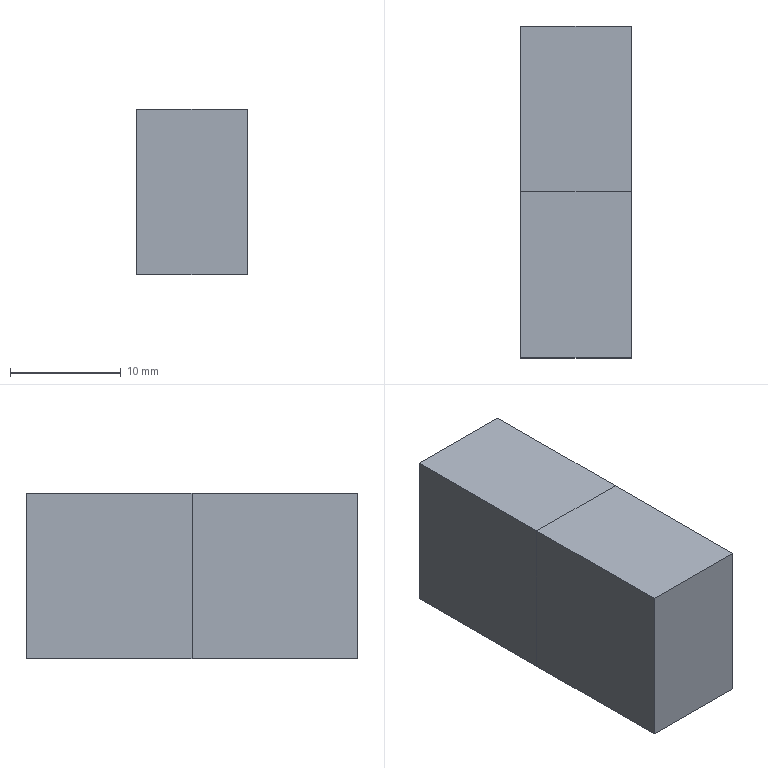Component | NX | 11_OBJECT | 2 solids | 12 faces | box 10 x 30 x 15 mm | volume 4500 mm3 | plane 12
STEP:
#1=CARTESIAN_POINT('',(0.,0.,0.));
#2=DIRECTION('',(0.,0.,1.));
#3=DIRECTION('',(1.,0.,0.));
#4=AXIS2_PLACEMENT_3D('',#1,#2,#3);
#5=CARTESIAN_POINT('',(2050.,126.,562.5));
#6=VERTEX_POINT('',#5);
#7=CARTESIAN_POINT('',(2050.,141.,562.5));
#8=VERTEX_POINT('',#7);
#9=CARTESIAN_POINT('',(2050.,126.,562.5));
#10=DIRECTION('',(0.,1.,0.));
#11=VECTOR('',#10,1.);
#12=LINE('',#9,#11);
#13=CARTESIAN_POINT('',(2060.,126.,562.5));
#14=DIRECTION('',(0.,0.,1.));
#15=DIRECTION('',(0.,1.,0.));
#16=AXIS2_PLACEMENT_3D('',#13,#14,#15);
#17=PLANE('',#16);
#18=CARTESIAN_POINT('',(0.,10.));
#19=DIRECTION('',(1.,0.));
#20=VECTOR('',#19,1.);
#21=LINE('',#18,#20);
#22=(GEOMETRIC_REPRESENTATION_CONTEXT(2)PARAMETRIC_REPRESENTATION_CONTEXT()REPRESENTATION_CONTEXT('',''));
#23=DEFINITIONAL_REPRESENTATION('',(#21),#22);
#24=PCURVE('',#17,#23);
#25=CARTESIAN_POINT('',(2050.,126.,562.5));
#26=DIRECTION('',(1.,0.,0.));
#27=DIRECTION('',(0.,1.,0.));
#28=AXIS2_PLACEMENT_3D('',#25,#26,#27);
#29=PLANE('',#28);
#30=CARTESIAN_POINT('',(0.,0.));
#31=DIRECTION('',(1.,0.));
#32=VECTOR('',#31,1.);
#33=LINE('',#30,#32);
#34=(GEOMETRIC_REPRESENTATION_CONTEXT(2)PARAMETRIC_REPRESENTATION_CONTEXT()REPRESENTATION_CONTEXT('',''));
#35=DEFINITIONAL_REPRESENTATION('',(#33),#34);
#36=PCURVE('',#29,#35);
#37=SURFACE_CURVE('',#12,(#24,#36),.PCURVE_S1.);
#38=EDGE_CURVE('',#6,#8,#37,.T.);
#39=ORIENTED_EDGE('',*,*,#38,.T.);
#40=CARTESIAN_POINT('',(2060.,141.,562.5));
#41=VERTEX_POINT('',#40);
#42=CARTESIAN_POINT('',(2060.,141.,562.5));
#43=DIRECTION('',(-1.,0.,0.));
#44=VECTOR('',#43,1.);
#45=LINE('',#42,#44);
#46=CARTESIAN_POINT('',(15.,0.));
#47=DIRECTION('',(0.,1.));
#48=VECTOR('',#47,1.);
#49=LINE('',#46,#48);
#50=(GEOMETRIC_REPRESENTATION_CONTEXT(2)PARAMETRIC_REPRESENTATION_CONTEXT()REPRESENTATION_CONTEXT('',''));
#51=DEFINITIONAL_REPRESENTATION('',(#49),#50);
#52=PCURVE('',#17,#51);
#53=CARTESIAN_POINT('',(2060.,141.,562.5));
#54=DIRECTION('',(0.,-1.,0.));
#55=DIRECTION('',(0.,0.,1.));
#56=AXIS2_PLACEMENT_3D('',#53,#54,#55);
#57=PLANE('',#56);
#58=CARTESIAN_POINT('',(0.,0.));
#59=DIRECTION('',(0.,1.));
#60=VECTOR('',#59,1.);
#61=LINE('',#58,#60);
#62=(GEOMETRIC_REPRESENTATION_CONTEXT(2)PARAMETRIC_REPRESENTATION_CONTEXT()REPRESENTATION_CONTEXT('',''));
#63=DEFINITIONAL_REPRESENTATION('',(#61),#62);
#64=PCURVE('',#57,#63);
#65=SURFACE_CURVE('',#45,(#52,#64),.PCURVE_S1.);
#66=EDGE_CURVE('',#41,#8,#65,.T.);
#67=ORIENTED_EDGE('',*,*,#66,.F.);
#68=CARTESIAN_POINT('',(2060.,126.,562.5));
#69=VERTEX_POINT('',#68);
#70=CARTESIAN_POINT('',(2060.,126.,562.5));
#71=DIRECTION('',(0.,1.,0.));
#72=VECTOR('',#71,1.);
#73=LINE('',#70,#72);
#74=CARTESIAN_POINT('',(0.,0.));
#75=DIRECTION('',(1.,0.));
#76=VECTOR('',#75,1.);
#77=LINE('',#74,#76);
#78=(GEOMETRIC_REPRESENTATION_CONTEXT(2)PARAMETRIC_REPRESENTATION_CONTEXT()REPRESENTATION_CONTEXT('',''));
#79=DEFINITIONAL_REPRESENTATION('',(#77),#78);
#80=PCURVE('',#17,#79);
#81=CARTESIAN_POINT('',(2060.,126.,562.5));
#82=DIRECTION('',(1.,0.,0.));
#83=DIRECTION('',(0.,1.,0.));
#84=AXIS2_PLACEMENT_3D('',#81,#82,#83);
#85=PLANE('',#84);
#86=CARTESIAN_POINT('',(0.,0.));
#87=DIRECTION('',(1.,0.));
#88=VECTOR('',#87,1.);
#89=LINE('',#86,#88);
#90=(GEOMETRIC_REPRESENTATION_CONTEXT(2)PARAMETRIC_REPRESENTATION_CONTEXT()REPRESENTATION_CONTEXT('',''));
#91=DEFINITIONAL_REPRESENTATION('',(#89),#90);
#92=PCURVE('',#85,#91);
#93=SURFACE_CURVE('',#73,(#80,#92),.PCURVE_S1.);
#94=EDGE_CURVE('',#69,#41,#93,.T.);
#95=ORIENTED_EDGE('',*,*,#94,.F.);
#96=CARTESIAN_POINT('',(2060.,126.,562.5));
#97=DIRECTION('',(-1.,0.,0.));
#98=VECTOR('',#97,1.);
#99=LINE('',#96,#98);
#100=CARTESIAN_POINT('',(0.,0.));
#101=DIRECTION('',(0.,1.));
#102=VECTOR('',#101,1.);
#103=LINE('',#100,#102);
#104=(GEOMETRIC_REPRESENTATION_CONTEXT(2)PARAMETRIC_REPRESENTATION_CONTEXT()REPRESENTATION_CONTEXT('',''));
#105=DEFINITIONAL_REPRESENTATION('',(#103),#104);
#106=PCURVE('',#17,#105);
#107=CARTESIAN_POINT('',(2060.,126.,577.5));
#108=DIRECTION('',(0.,1.,0.));
#109=DIRECTION('',(0.,0.,-1.));
#110=AXIS2_PLACEMENT_3D('',#107,#108,#109);
#111=PLANE('',#110);
#112=CARTESIAN_POINT('',(15.,0.));
#113=DIRECTION('',(0.,1.));
#114=VECTOR('',#113,1.);
#115=LINE('',#112,#114);
#116=(GEOMETRIC_REPRESENTATION_CONTEXT(2)PARAMETRIC_REPRESENTATION_CONTEXT()REPRESENTATION_CONTEXT('',''));
#117=DEFINITIONAL_REPRESENTATION('',(#115),#116);
#118=PCURVE('',#111,#117);
#119=SURFACE_CURVE('',#99,(#106,#118),.PCURVE_S1.);
#120=EDGE_CURVE('',#69,#6,#119,.T.);
#121=ORIENTED_EDGE('',*,*,#120,.T.);
#122=EDGE_LOOP('',(#39,#67,#95,#121));
#123=FACE_BOUND('',#122,.T.);
#124=ADVANCED_FACE('',(#123),#17,.F.);
#125=CARTESIAN_POINT('',(2050.,141.,577.5));
#126=VERTEX_POINT('',#125);
#127=CARTESIAN_POINT('',(2050.,141.,562.5));
#128=DIRECTION('',(0.,0.,1.));
#129=VECTOR('',#128,1.);
#130=LINE('',#127,#129);
#131=CARTESIAN_POINT('',(0.,10.));
#132=DIRECTION('',(1.,0.));
#133=VECTOR('',#132,1.);
#134=LINE('',#131,#133);
#135=(GEOMETRIC_REPRESENTATION_CONTEXT(2)PARAMETRIC_REPRESENTATION_CONTEXT()REPRESENTATION_CONTEXT('',''));
#136=DEFINITIONAL_REPRESENTATION('',(#134),#135);
#137=PCURVE('',#57,#136);
#138=CARTESIAN_POINT('',(15.,0.));
#139=DIRECTION('',(0.,1.));
#140=VECTOR('',#139,1.);
#141=LINE('',#138,#140);
#142=(GEOMETRIC_REPRESENTATION_CONTEXT(2)PARAMETRIC_REPRESENTATION_CONTEXT()REPRESENTATION_CONTEXT('',''));
#143=DEFINITIONAL_REPRESENTATION('',(#141),#142);
#144=PCURVE('',#29,#143);
#145=SURFACE_CURVE('',#130,(#137,#144),.PCURVE_S1.);
#146=EDGE_CURVE('',#8,#126,#145,.T.);
#147=ORIENTED_EDGE('',*,*,#146,.T.);
#148=CARTESIAN_POINT('',(2060.,141.,577.5));
#149=VERTEX_POINT('',#148);
#150=CARTESIAN_POINT('',(2060.,141.,577.5));
#151=DIRECTION('',(-1.,0.,0.));
#152=VECTOR('',#151,1.);
#153=LINE('',#150,#152);
#154=CARTESIAN_POINT('',(15.,0.));
#155=DIRECTION('',(0.,1.));
#156=VECTOR('',#155,1.);
#157=LINE('',#154,#156);
#158=(GEOMETRIC_REPRESENTATION_CONTEXT(2)PARAMETRIC_REPRESENTATION_CONTEXT()REPRESENTATION_CONTEXT('',''));
#159=DEFINITIONAL_REPRESENTATION('',(#157),#158);
#160=PCURVE('',#57,#159);
#161=CARTESIAN_POINT('',(2060.,141.,577.5));
#162=DIRECTION('',(0.,0.,-1.));
#163=DIRECTION('',(0.,-1.,0.));
#164=AXIS2_PLACEMENT_3D('',#161,#162,#163);
#165=PLANE('',#164);
#166=CARTESIAN_POINT('',(0.,0.));
#167=DIRECTION('',(0.,1.));
#168=VECTOR('',#167,1.);
#169=LINE('',#166,#168);
#170=(GEOMETRIC_REPRESENTATION_CONTEXT(2)PARAMETRIC_REPRESENTATION_CONTEXT()REPRESENTATION_CONTEXT('',''));
#171=DEFINITIONAL_REPRESENTATION('',(#169),#170);
#172=PCURVE('',#165,#171);
#173=SURFACE_CURVE('',#153,(#160,#172),.PCURVE_S1.);
#174=EDGE_CURVE('',#149,#126,#173,.T.);
#175=ORIENTED_EDGE('',*,*,#174,.F.);
#176=CARTESIAN_POINT('',(2060.,141.,562.5));
#177=DIRECTION('',(0.,0.,1.));
#178=VECTOR('',#177,1.);
#179=LINE('',#176,#178);
#180=CARTESIAN_POINT('',(0.,0.));
#181=DIRECTION('',(1.,0.));
#182=VECTOR('',#181,1.);
#183=LINE('',#180,#182);
#184=(GEOMETRIC_REPRESENTATION_CONTEXT(2)PARAMETRIC_REPRESENTATION_CONTEXT()REPRESENTATION_CONTEXT('',''));
#185=DEFINITIONAL_REPRESENTATION('',(#183),#184);
#186=PCURVE('',#57,#185);
#187=CARTESIAN_POINT('',(15.,0.));
#188=DIRECTION('',(0.,1.));
#189=VECTOR('',#188,1.);
#190=LINE('',#187,#189);
#191=(GEOMETRIC_REPRESENTATION_CONTEXT(2)PARAMETRIC_REPRESENTATION_CONTEXT()REPRESENTATION_CONTEXT('',''));
#192=DEFINITIONAL_REPRESENTATION('',(#190),#191);
#193=PCURVE('',#85,#192);
#194=SURFACE_CURVE('',#179,(#186,#193),.PCURVE_S1.);
#195=EDGE_CURVE('',#41,#149,#194,.T.);
#196=ORIENTED_EDGE('',*,*,#195,.F.);
#197=ORIENTED_EDGE('',*,*,#66,.T.);
#198=EDGE_LOOP('',(#147,#175,#196,#197));
#199=FACE_BOUND('',#198,.T.);
#200=ADVANCED_FACE('',(#199),#57,.F.);
#201=CARTESIAN_POINT('',(2050.,126.,577.5));
#202=VERTEX_POINT('',#201);
#203=CARTESIAN_POINT('',(2050.,141.,577.5));
#204=DIRECTION('',(0.,-1.,0.));
#205=VECTOR('',#204,1.);
#206=LINE('',#203,#205);
#207=CARTESIAN_POINT('',(0.,10.));
#208=DIRECTION('',(1.,0.));
#209=VECTOR('',#208,1.);
#210=LINE('',#207,#209);
#211=(GEOMETRIC_REPRESENTATION_CONTEXT(2)PARAMETRIC_REPRESENTATION_CONTEXT()REPRESENTATION_CONTEXT('',''));
#212=DEFINITIONAL_REPRESENTATION('',(#210),#211);
#213=PCURVE('',#165,#212);
#214=CARTESIAN_POINT('',(15.,15.));
#215=DIRECTION('',(-1.,0.));
#216=VECTOR('',#215,1.);
#217=LINE('',#214,#216);
#218=(GEOMETRIC_REPRESENTATION_CONTEXT(2)PARAMETRIC_REPRESENTATION_CONTEXT()REPRESENTATION_CONTEXT('',''));
#219=DEFINITIONAL_REPRESENTATION('',(#217),#218);
#220=PCURVE('',#29,#219);
#221=SURFACE_CURVE('',#206,(#213,#220),.PCURVE_S1.);
#222=EDGE_CURVE('',#126,#202,#221,.T.);
#223=ORIENTED_EDGE('',*,*,#222,.T.);
#224=CARTESIAN_POINT('',(2060.,126.,577.5));
#225=VERTEX_POINT('',#224);
#226=CARTESIAN_POINT('',(2060.,126.,577.5));
#227=DIRECTION('',(-1.,0.,0.));
#228=VECTOR('',#227,1.);
#229=LINE('',#226,#228);
#230=CARTESIAN_POINT('',(15.,0.));
#231=DIRECTION('',(0.,1.));
#232=VECTOR('',#231,1.);
#233=LINE('',#230,#232);
#234=(GEOMETRIC_REPRESENTATION_CONTEXT(2)PARAMETRIC_REPRESENTATION_CONTEXT()REPRESENTATION_CONTEXT('',''));
#235=DEFINITIONAL_REPRESENTATION('',(#233),#234);
#236=PCURVE('',#165,#235);
#237=CARTESIAN_POINT('',(0.,0.));
#238=DIRECTION('',(0.,1.));
#239=VECTOR('',#238,1.);
#240=LINE('',#237,#239);
#241=(GEOMETRIC_REPRESENTATION_CONTEXT(2)PARAMETRIC_REPRESENTATION_CONTEXT()REPRESENTATION_CONTEXT('',''));
#242=DEFINITIONAL_REPRESENTATION('',(#240),#241);
#243=PCURVE('',#111,#242);
#244=SURFACE_CURVE('',#229,(#236,#243),.PCURVE_S1.);
#245=EDGE_CURVE('',#225,#202,#244,.T.);
#246=ORIENTED_EDGE('',*,*,#245,.F.);
#247=CARTESIAN_POINT('',(2060.,141.,577.5));
#248=DIRECTION('',(0.,-1.,0.));
#249=VECTOR('',#248,1.);
#250=LINE('',#247,#249);
#251=CARTESIAN_POINT('',(0.,0.));
#252=DIRECTION('',(1.,0.));
#253=VECTOR('',#252,1.);
#254=LINE('',#251,#253);
#255=(GEOMETRIC_REPRESENTATION_CONTEXT(2)PARAMETRIC_REPRESENTATION_CONTEXT()REPRESENTATION_CONTEXT('',''));
#256=DEFINITIONAL_REPRESENTATION('',(#254),#255);
#257=PCURVE('',#165,#256);
#258=CARTESIAN_POINT('',(15.,15.));
#259=DIRECTION('',(-1.,0.));
#260=VECTOR('',#259,1.);
#261=LINE('',#258,#260);
#262=(GEOMETRIC_REPRESENTATION_CONTEXT(2)PARAMETRIC_REPRESENTATION_CONTEXT()REPRESENTATION_CONTEXT('',''));
#263=DEFINITIONAL_REPRESENTATION('',(#261),#262);
#264=PCURVE('',#85,#263);
#265=SURFACE_CURVE('',#250,(#257,#264),.PCURVE_S1.);
#266=EDGE_CURVE('',#149,#225,#265,.T.);
#267=ORIENTED_EDGE('',*,*,#266,.F.);
#268=ORIENTED_EDGE('',*,*,#174,.T.);
#269=EDGE_LOOP('',(#223,#246,#267,#268));
#270=FACE_BOUND('',#269,.T.);
#271=ADVANCED_FACE('',(#270),#165,.F.);
#272=CARTESIAN_POINT('',(2050.,126.,577.5));
#273=DIRECTION('',(0.,0.,-1.));
#274=VECTOR('',#273,1.);
#275=LINE('',#272,#274);
#276=CARTESIAN_POINT('',(0.,10.));
#277=DIRECTION('',(1.,0.));
#278=VECTOR('',#277,1.);
#279=LINE('',#276,#278);
#280=(GEOMETRIC_REPRESENTATION_CONTEXT(2)PARAMETRIC_REPRESENTATION_CONTEXT()REPRESENTATION_CONTEXT('',''));
#281=DEFINITIONAL_REPRESENTATION('',(#279),#280);
#282=PCURVE('',#111,#281);
#283=CARTESIAN_POINT('',(0.,15.));
#284=DIRECTION('',(0.,-1.));
#285=VECTOR('',#284,1.);
#286=LINE('',#283,#285);
#287=(GEOMETRIC_REPRESENTATION_CONTEXT(2)PARAMETRIC_REPRESENTATION_CONTEXT()REPRESENTATION_CONTEXT('',''));
#288=DEFINITIONAL_REPRESENTATION('',(#286),#287);
#289=PCURVE('',#29,#288);
#290=SURFACE_CURVE('',#275,(#282,#289),.PCURVE_S1.);
#291=EDGE_CURVE('',#202,#6,#290,.T.);
#292=ORIENTED_EDGE('',*,*,#291,.T.);
#293=ORIENTED_EDGE('',*,*,#120,.F.);
#294=CARTESIAN_POINT('',(2060.,126.,577.5));
#295=DIRECTION('',(0.,0.,-1.));
#296=VECTOR('',#295,1.);
#297=LINE('',#294,#296);
#298=CARTESIAN_POINT('',(0.,0.));
#299=DIRECTION('',(1.,0.));
#300=VECTOR('',#299,1.);
#301=LINE('',#298,#300);
#302=(GEOMETRIC_REPRESENTATION_CONTEXT(2)PARAMETRIC_REPRESENTATION_CONTEXT()REPRESENTATION_CONTEXT('',''));
#303=DEFINITIONAL_REPRESENTATION('',(#301),#302);
#304=PCURVE('',#111,#303);
#305=CARTESIAN_POINT('',(0.,15.));
#306=DIRECTION('',(0.,-1.));
#307=VECTOR('',#306,1.);
#308=LINE('',#305,#307);
#309=(GEOMETRIC_REPRESENTATION_CONTEXT(2)PARAMETRIC_REPRESENTATION_CONTEXT()REPRESENTATION_CONTEXT('',''));
#310=DEFINITIONAL_REPRESENTATION('',(#308),#309);
#311=PCURVE('',#85,#310);
#312=SURFACE_CURVE('',#297,(#304,#311),.PCURVE_S1.);
#313=EDGE_CURVE('',#225,#69,#312,.T.);
#314=ORIENTED_EDGE('',*,*,#313,.F.);
#315=ORIENTED_EDGE('',*,*,#245,.T.);
#316=EDGE_LOOP('',(#292,#293,#314,#315));
#317=FACE_BOUND('',#316,.T.);
#318=ADVANCED_FACE('',(#317),#111,.F.);
#319=ORIENTED_EDGE('',*,*,#94,.T.);
#320=ORIENTED_EDGE('',*,*,#195,.T.);
#321=ORIENTED_EDGE('',*,*,#266,.T.);
#322=ORIENTED_EDGE('',*,*,#313,.T.);
#323=EDGE_LOOP('',(#319,#320,#321,#322));
#324=FACE_BOUND('',#323,.T.);
#325=ADVANCED_FACE('',(#324),#85,.T.);
#326=ORIENTED_EDGE('',*,*,#38,.F.);
#327=ORIENTED_EDGE('',*,*,#291,.F.);
#328=ORIENTED_EDGE('',*,*,#222,.F.);
#329=ORIENTED_EDGE('',*,*,#146,.F.);
#330=EDGE_LOOP('',(#326,#327,#328,#329));
#331=FACE_BOUND('',#330,.T.);
#332=ADVANCED_FACE('',(#331),#29,.F.);
#333=CLOSED_SHELL('',(#124,#200,#271,#318,#325,#332));
#334=MANIFOLD_SOLID_BREP('',#333);
#335=(LENGTH_UNIT()NAMED_UNIT(*)SI_UNIT(.MILLI.,.METRE.));
#336=UNCERTAINTY_MEASURE_WITH_UNIT(LENGTH_MEASURE(0.0000001),#335,'','');
#337=(NAMED_UNIT(*)PLANE_ANGLE_UNIT()SI_UNIT($,.RADIAN.));
#338=(NAMED_UNIT(*)SI_UNIT($,.STERADIAN.)SOLID_ANGLE_UNIT());
#339=(GEOMETRIC_REPRESENTATION_CONTEXT(3)GLOBAL_UNCERTAINTY_ASSIGNED_CONTEXT((#336))GLOBAL_UNIT_ASSIGNED_CONTEXT((#335,#337,#338))REPRESENTATION_CONTEXT('',''));
#340=ADVANCED_BREP_SHAPE_REPRESENTATION('',(#4,#334),#339);
#341=CARTESIAN_POINT('',(0.,0.,0.));
#342=DIRECTION('',(0.,0.,1.));
#343=DIRECTION('',(1.,0.,0.));
#344=AXIS2_PLACEMENT_3D('',#341,#342,#343);
#345=CARTESIAN_POINT('',(0.,0.,0.));
#346=DIRECTION('',(0.,0.,1.));
#347=DIRECTION('',(1.,0.,0.));
#348=AXIS2_PLACEMENT_3D('',#345,#346,#347);
#349=(LENGTH_UNIT()NAMED_UNIT(*)SI_UNIT(.MILLI.,.METRE.));
#350=UNCERTAINTY_MEASURE_WITH_UNIT(LENGTH_MEASURE(0.0000001),#349,'','');
#351=(NAMED_UNIT(*)PLANE_ANGLE_UNIT()SI_UNIT($,.RADIAN.));
#352=(NAMED_UNIT(*)SI_UNIT($,.STERADIAN.)SOLID_ANGLE_UNIT());
#353=(GEOMETRIC_REPRESENTATION_CONTEXT(3)GLOBAL_UNCERTAINTY_ASSIGNED_CONTEXT((#350))GLOBAL_UNIT_ASSIGNED_CONTEXT((#349,#351,#352))REPRESENTATION_CONTEXT('',''));
#354=SHAPE_REPRESENTATION('',(#4,#344,#348),#353);
#355=ITEM_DEFINED_TRANSFORMATION('','',#4,#344);
#356=(REPRESENTATION_RELATIONSHIP('','',#340,#354)REPRESENTATION_RELATIONSHIP_WITH_TRANSFORMATION(#355)SHAPE_REPRESENTATION_RELATIONSHIP());
#357=CARTESIAN_POINT('',(2050.,111.,562.5));
#358=VERTEX_POINT('',#357);
#359=CARTESIAN_POINT('',(2050.,126.,562.5));
#360=VERTEX_POINT('',#359);
#361=CARTESIAN_POINT('',(2050.,111.,562.5));
#362=DIRECTION('',(0.,1.,0.));
#363=VECTOR('',#362,1.);
#364=LINE('',#361,#363);
#365=CARTESIAN_POINT('',(2060.,111.,562.5));
#366=DIRECTION('',(0.,0.,1.));
#367=DIRECTION('',(0.,1.,0.));
#368=AXIS2_PLACEMENT_3D('',#365,#366,#367);
#369=PLANE('',#368);
#370=CARTESIAN_POINT('',(0.,10.));
#371=DIRECTION('',(1.,0.));
#372=VECTOR('',#371,1.);
#373=LINE('',#370,#372);
#374=(GEOMETRIC_REPRESENTATION_CONTEXT(2)PARAMETRIC_REPRESENTATION_CONTEXT()REPRESENTATION_CONTEXT('',''));
#375=DEFINITIONAL_REPRESENTATION('',(#373),#374);
#376=PCURVE('',#369,#375);
#377=CARTESIAN_POINT('',(2050.,111.,562.5));
#378=DIRECTION('',(1.,0.,0.));
#379=DIRECTION('',(0.,1.,0.));
#380=AXIS2_PLACEMENT_3D('',#377,#378,#379);
#381=PLANE('',#380);
#382=CARTESIAN_POINT('',(0.,0.));
#383=DIRECTION('',(1.,0.));
#384=VECTOR('',#383,1.);
#385=LINE('',#382,#384);
#386=(GEOMETRIC_REPRESENTATION_CONTEXT(2)PARAMETRIC_REPRESENTATION_CONTEXT()REPRESENTATION_CONTEXT('',''));
#387=DEFINITIONAL_REPRESENTATION('',(#385),#386);
#388=PCURVE('',#381,#387);
#389=SURFACE_CURVE('',#364,(#376,#388),.PCURVE_S1.);
#390=EDGE_CURVE('',#358,#360,#389,.T.);
#391=ORIENTED_EDGE('',*,*,#390,.T.);
#392=CARTESIAN_POINT('',(2060.,126.,562.5));
#393=VERTEX_POINT('',#392);
#394=CARTESIAN_POINT('',(2060.,126.,562.5));
#395=DIRECTION('',(-1.,0.,0.));
#396=VECTOR('',#395,1.);
#397=LINE('',#394,#396);
#398=CARTESIAN_POINT('',(15.,0.));
#399=DIRECTION('',(0.,1.));
#400=VECTOR('',#399,1.);
#401=LINE('',#398,#400);
#402=(GEOMETRIC_REPRESENTATION_CONTEXT(2)PARAMETRIC_REPRESENTATION_CONTEXT()REPRESENTATION_CONTEXT('',''));
#403=DEFINITIONAL_REPRESENTATION('',(#401),#402);
#404=PCURVE('',#369,#403);
#405=CARTESIAN_POINT('',(2060.,126.,562.5));
#406=DIRECTION('',(0.,-1.,0.));
#407=DIRECTION('',(0.,0.,1.));
#408=AXIS2_PLACEMENT_3D('',#405,#406,#407);
#409=PLANE('',#408);
#410=CARTESIAN_POINT('',(0.,0.));
#411=DIRECTION('',(0.,1.));
#412=VECTOR('',#411,1.);
#413=LINE('',#410,#412);
#414=(GEOMETRIC_REPRESENTATION_CONTEXT(2)PARAMETRIC_REPRESENTATION_CONTEXT()REPRESENTATION_CONTEXT('',''));
#415=DEFINITIONAL_REPRESENTATION('',(#413),#414);
#416=PCURVE('',#409,#415);
#417=SURFACE_CURVE('',#397,(#404,#416),.PCURVE_S1.);
#418=EDGE_CURVE('',#393,#360,#417,.T.);
#419=ORIENTED_EDGE('',*,*,#418,.F.);
#420=CARTESIAN_POINT('',(2060.,111.,562.5));
#421=VERTEX_POINT('',#420);
#422=CARTESIAN_POINT('',(2060.,111.,562.5));
#423=DIRECTION('',(0.,1.,0.));
#424=VECTOR('',#423,1.);
#425=LINE('',#422,#424);
#426=CARTESIAN_POINT('',(0.,0.));
#427=DIRECTION('',(1.,0.));
#428=VECTOR('',#427,1.);
#429=LINE('',#426,#428);
#430=(GEOMETRIC_REPRESENTATION_CONTEXT(2)PARAMETRIC_REPRESENTATION_CONTEXT()REPRESENTATION_CONTEXT('',''));
#431=DEFINITIONAL_REPRESENTATION('',(#429),#430);
#432=PCURVE('',#369,#431);
#433=CARTESIAN_POINT('',(2060.,111.,562.5));
#434=DIRECTION('',(1.,0.,0.));
#435=DIRECTION('',(0.,1.,0.));
#436=AXIS2_PLACEMENT_3D('',#433,#434,#435);
#437=PLANE('',#436);
#438=CARTESIAN_POINT('',(0.,0.));
#439=DIRECTION('',(1.,0.));
#440=VECTOR('',#439,1.);
#441=LINE('',#438,#440);
#442=(GEOMETRIC_REPRESENTATION_CONTEXT(2)PARAMETRIC_REPRESENTATION_CONTEXT()REPRESENTATION_CONTEXT('',''));
#443=DEFINITIONAL_REPRESENTATION('',(#441),#442);
#444=PCURVE('',#437,#443);
#445=SURFACE_CURVE('',#425,(#432,#444),.PCURVE_S1.);
#446=EDGE_CURVE('',#421,#393,#445,.T.);
#447=ORIENTED_EDGE('',*,*,#446,.F.);
#448=CARTESIAN_POINT('',(2060.,111.,562.5));
#449=DIRECTION('',(-1.,0.,0.));
#450=VECTOR('',#449,1.);
#451=LINE('',#448,#450);
#452=CARTESIAN_POINT('',(0.,0.));
#453=DIRECTION('',(0.,1.));
#454=VECTOR('',#453,1.);
#455=LINE('',#452,#454);
#456=(GEOMETRIC_REPRESENTATION_CONTEXT(2)PARAMETRIC_REPRESENTATION_CONTEXT()REPRESENTATION_CONTEXT('',''));
#457=DEFINITIONAL_REPRESENTATION('',(#455),#456);
#458=PCURVE('',#369,#457);
#459=CARTESIAN_POINT('',(2060.,111.,577.5));
#460=DIRECTION('',(0.,1.,0.));
#461=DIRECTION('',(0.,0.,-1.));
#462=AXIS2_PLACEMENT_3D('',#459,#460,#461);
#463=PLANE('',#462);
#464=CARTESIAN_POINT('',(15.,0.));
#465=DIRECTION('',(0.,1.));
#466=VECTOR('',#465,1.);
#467=LINE('',#464,#466);
#468=(GEOMETRIC_REPRESENTATION_CONTEXT(2)PARAMETRIC_REPRESENTATION_CONTEXT()REPRESENTATION_CONTEXT('',''));
#469=DEFINITIONAL_REPRESENTATION('',(#467),#468);
#470=PCURVE('',#463,#469);
#471=SURFACE_CURVE('',#451,(#458,#470),.PCURVE_S1.);
#472=EDGE_CURVE('',#421,#358,#471,.T.);
#473=ORIENTED_EDGE('',*,*,#472,.T.);
#474=EDGE_LOOP('',(#391,#419,#447,#473));
#475=FACE_BOUND('',#474,.T.);
#476=ADVANCED_FACE('',(#475),#369,.F.);
#477=CARTESIAN_POINT('',(2050.,126.,577.5));
#478=VERTEX_POINT('',#477);
#479=CARTESIAN_POINT('',(2050.,126.,562.5));
#480=DIRECTION('',(0.,0.,1.));
#481=VECTOR('',#480,1.);
#482=LINE('',#479,#481);
#483=CARTESIAN_POINT('',(0.,10.));
#484=DIRECTION('',(1.,0.));
#485=VECTOR('',#484,1.);
#486=LINE('',#483,#485);
#487=(GEOMETRIC_REPRESENTATION_CONTEXT(2)PARAMETRIC_REPRESENTATION_CONTEXT()REPRESENTATION_CONTEXT('',''));
#488=DEFINITIONAL_REPRESENTATION('',(#486),#487);
#489=PCURVE('',#409,#488);
#490=CARTESIAN_POINT('',(15.,0.));
#491=DIRECTION('',(0.,1.));
#492=VECTOR('',#491,1.);
#493=LINE('',#490,#492);
#494=(GEOMETRIC_REPRESENTATION_CONTEXT(2)PARAMETRIC_REPRESENTATION_CONTEXT()REPRESENTATION_CONTEXT('',''));
#495=DEFINITIONAL_REPRESENTATION('',(#493),#494);
#496=PCURVE('',#381,#495);
#497=SURFACE_CURVE('',#482,(#489,#496),.PCURVE_S1.);
#498=EDGE_CURVE('',#360,#478,#497,.T.);
#499=ORIENTED_EDGE('',*,*,#498,.T.);
#500=CARTESIAN_POINT('',(2060.,126.,577.5));
#501=VERTEX_POINT('',#500);
#502=CARTESIAN_POINT('',(2060.,126.,577.5));
#503=DIRECTION('',(-1.,0.,0.));
#504=VECTOR('',#503,1.);
#505=LINE('',#502,#504);
#506=CARTESIAN_POINT('',(15.,0.));
#507=DIRECTION('',(0.,1.));
#508=VECTOR('',#507,1.);
#509=LINE('',#506,#508);
#510=(GEOMETRIC_REPRESENTATION_CONTEXT(2)PARAMETRIC_REPRESENTATION_CONTEXT()REPRESENTATION_CONTEXT('',''));
#511=DEFINITIONAL_REPRESENTATION('',(#509),#510);
#512=PCURVE('',#409,#511);
#513=CARTESIAN_POINT('',(2060.,126.,577.5));
#514=DIRECTION('',(0.,0.,-1.));
#515=DIRECTION('',(0.,-1.,0.));
#516=AXIS2_PLACEMENT_3D('',#513,#514,#515);
#517=PLANE('',#516);
#518=CARTESIAN_POINT('',(0.,0.));
#519=DIRECTION('',(0.,1.));
#520=VECTOR('',#519,1.);
#521=LINE('',#518,#520);
#522=(GEOMETRIC_REPRESENTATION_CONTEXT(2)PARAMETRIC_REPRESENTATION_CONTEXT()REPRESENTATION_CONTEXT('',''));
#523=DEFINITIONAL_REPRESENTATION('',(#521),#522);
#524=PCURVE('',#517,#523);
#525=SURFACE_CURVE('',#505,(#512,#524),.PCURVE_S1.);
#526=EDGE_CURVE('',#501,#478,#525,.T.);
#527=ORIENTED_EDGE('',*,*,#526,.F.);
#528=CARTESIAN_POINT('',(2060.,126.,562.5));
#529=DIRECTION('',(0.,0.,1.));
#530=VECTOR('',#529,1.);
#531=LINE('',#528,#530);
#532=CARTESIAN_POINT('',(0.,0.));
#533=DIRECTION('',(1.,0.));
#534=VECTOR('',#533,1.);
#535=LINE('',#532,#534);
#536=(GEOMETRIC_REPRESENTATION_CONTEXT(2)PARAMETRIC_REPRESENTATION_CONTEXT()REPRESENTATION_CONTEXT('',''));
#537=DEFINITIONAL_REPRESENTATION('',(#535),#536);
#538=PCURVE('',#409,#537);
#539=CARTESIAN_POINT('',(15.,0.));
#540=DIRECTION('',(0.,1.));
#541=VECTOR('',#540,1.);
#542=LINE('',#539,#541);
#543=(GEOMETRIC_REPRESENTATION_CONTEXT(2)PARAMETRIC_REPRESENTATION_CONTEXT()REPRESENTATION_CONTEXT('',''));
#544=DEFINITIONAL_REPRESENTATION('',(#542),#543);
#545=PCURVE('',#437,#544);
#546=SURFACE_CURVE('',#531,(#538,#545),.PCURVE_S1.);
#547=EDGE_CURVE('',#393,#501,#546,.T.);
#548=ORIENTED_EDGE('',*,*,#547,.F.);
#549=ORIENTED_EDGE('',*,*,#418,.T.);
#550=EDGE_LOOP('',(#499,#527,#548,#549));
#551=FACE_BOUND('',#550,.T.);
#552=ADVANCED_FACE('',(#551),#409,.F.);
#553=CARTESIAN_POINT('',(2050.,111.,577.5));
#554=VERTEX_POINT('',#553);
#555=CARTESIAN_POINT('',(2050.,126.,577.5));
#556=DIRECTION('',(0.,-1.,0.));
#557=VECTOR('',#556,1.);
#558=LINE('',#555,#557);
#559=CARTESIAN_POINT('',(0.,10.));
#560=DIRECTION('',(1.,0.));
#561=VECTOR('',#560,1.);
#562=LINE('',#559,#561);
#563=(GEOMETRIC_REPRESENTATION_CONTEXT(2)PARAMETRIC_REPRESENTATION_CONTEXT()REPRESENTATION_CONTEXT('',''));
#564=DEFINITIONAL_REPRESENTATION('',(#562),#563);
#565=PCURVE('',#517,#564);
#566=CARTESIAN_POINT('',(15.,15.));
#567=DIRECTION('',(-1.,0.));
#568=VECTOR('',#567,1.);
#569=LINE('',#566,#568);
#570=(GEOMETRIC_REPRESENTATION_CONTEXT(2)PARAMETRIC_REPRESENTATION_CONTEXT()REPRESENTATION_CONTEXT('',''));
#571=DEFINITIONAL_REPRESENTATION('',(#569),#570);
#572=PCURVE('',#381,#571);
#573=SURFACE_CURVE('',#558,(#565,#572),.PCURVE_S1.);
#574=EDGE_CURVE('',#478,#554,#573,.T.);
#575=ORIENTED_EDGE('',*,*,#574,.T.);
#576=CARTESIAN_POINT('',(2060.,111.,577.5));
#577=VERTEX_POINT('',#576);
#578=CARTESIAN_POINT('',(2060.,111.,577.5));
#579=DIRECTION('',(-1.,0.,0.));
#580=VECTOR('',#579,1.);
#581=LINE('',#578,#580);
#582=CARTESIAN_POINT('',(15.,0.));
#583=DIRECTION('',(0.,1.));
#584=VECTOR('',#583,1.);
#585=LINE('',#582,#584);
#586=(GEOMETRIC_REPRESENTATION_CONTEXT(2)PARAMETRIC_REPRESENTATION_CONTEXT()REPRESENTATION_CONTEXT('',''));
#587=DEFINITIONAL_REPRESENTATION('',(#585),#586);
#588=PCURVE('',#517,#587);
#589=CARTESIAN_POINT('',(0.,0.));
#590=DIRECTION('',(0.,1.));
#591=VECTOR('',#590,1.);
#592=LINE('',#589,#591);
#593=(GEOMETRIC_REPRESENTATION_CONTEXT(2)PARAMETRIC_REPRESENTATION_CONTEXT()REPRESENTATION_CONTEXT('',''));
#594=DEFINITIONAL_REPRESENTATION('',(#592),#593);
#595=PCURVE('',#463,#594);
#596=SURFACE_CURVE('',#581,(#588,#595),.PCURVE_S1.);
#597=EDGE_CURVE('',#577,#554,#596,.T.);
#598=ORIENTED_EDGE('',*,*,#597,.F.);
#599=CARTESIAN_POINT('',(2060.,126.,577.5));
#600=DIRECTION('',(0.,-1.,0.));
#601=VECTOR('',#600,1.);
#602=LINE('',#599,#601);
#603=CARTESIAN_POINT('',(0.,0.));
#604=DIRECTION('',(1.,0.));
#605=VECTOR('',#604,1.);
#606=LINE('',#603,#605);
#607=(GEOMETRIC_REPRESENTATION_CONTEXT(2)PARAMETRIC_REPRESENTATION_CONTEXT()REPRESENTATION_CONTEXT('',''));
#608=DEFINITIONAL_REPRESENTATION('',(#606),#607);
#609=PCURVE('',#517,#608);
#610=CARTESIAN_POINT('',(15.,15.));
#611=DIRECTION('',(-1.,0.));
#612=VECTOR('',#611,1.);
#613=LINE('',#610,#612);
#614=(GEOMETRIC_REPRESENTATION_CONTEXT(2)PARAMETRIC_REPRESENTATION_CONTEXT()REPRESENTATION_CONTEXT('',''));
#615=DEFINITIONAL_REPRESENTATION('',(#613),#614);
#616=PCURVE('',#437,#615);
#617=SURFACE_CURVE('',#602,(#609,#616),.PCURVE_S1.);
#618=EDGE_CURVE('',#501,#577,#617,.T.);
#619=ORIENTED_EDGE('',*,*,#618,.F.);
#620=ORIENTED_EDGE('',*,*,#526,.T.);
#621=EDGE_LOOP('',(#575,#598,#619,#620));
#622=FACE_BOUND('',#621,.T.);
#623=ADVANCED_FACE('',(#622),#517,.F.);
#624=CARTESIAN_POINT('',(2050.,111.,577.5));
#625=DIRECTION('',(0.,0.,-1.));
#626=VECTOR('',#625,1.);
#627=LINE('',#624,#626);
#628=CARTESIAN_POINT('',(0.,10.));
#629=DIRECTION('',(1.,0.));
#630=VECTOR('',#629,1.);
#631=LINE('',#628,#630);
#632=(GEOMETRIC_REPRESENTATION_CONTEXT(2)PARAMETRIC_REPRESENTATION_CONTEXT()REPRESENTATION_CONTEXT('',''));
#633=DEFINITIONAL_REPRESENTATION('',(#631),#632);
#634=PCURVE('',#463,#633);
#635=CARTESIAN_POINT('',(0.,15.));
#636=DIRECTION('',(0.,-1.));
#637=VECTOR('',#636,1.);
#638=LINE('',#635,#637);
#639=(GEOMETRIC_REPRESENTATION_CONTEXT(2)PARAMETRIC_REPRESENTATION_CONTEXT()REPRESENTATION_CONTEXT('',''));
#640=DEFINITIONAL_REPRESENTATION('',(#638),#639);
#641=PCURVE('',#381,#640);
#642=SURFACE_CURVE('',#627,(#634,#641),.PCURVE_S1.);
#643=EDGE_CURVE('',#554,#358,#642,.T.);
#644=ORIENTED_EDGE('',*,*,#643,.T.);
#645=ORIENTED_EDGE('',*,*,#472,.F.);
#646=CARTESIAN_POINT('',(2060.,111.,577.5));
#647=DIRECTION('',(0.,0.,-1.));
#648=VECTOR('',#647,1.);
#649=LINE('',#646,#648);
#650=CARTESIAN_POINT('',(0.,0.));
#651=DIRECTION('',(1.,0.));
#652=VECTOR('',#651,1.);
#653=LINE('',#650,#652);
#654=(GEOMETRIC_REPRESENTATION_CONTEXT(2)PARAMETRIC_REPRESENTATION_CONTEXT()REPRESENTATION_CONTEXT('',''));
#655=DEFINITIONAL_REPRESENTATION('',(#653),#654);
#656=PCURVE('',#463,#655);
#657=CARTESIAN_POINT('',(0.,15.));
#658=DIRECTION('',(0.,-1.));
#659=VECTOR('',#658,1.);
#660=LINE('',#657,#659);
#661=(GEOMETRIC_REPRESENTATION_CONTEXT(2)PARAMETRIC_REPRESENTATION_CONTEXT()REPRESENTATION_CONTEXT('',''));
#662=DEFINITIONAL_REPRESENTATION('',(#660),#661);
#663=PCURVE('',#437,#662);
#664=SURFACE_CURVE('',#649,(#656,#663),.PCURVE_S1.);
#665=EDGE_CURVE('',#577,#421,#664,.T.);
#666=ORIENTED_EDGE('',*,*,#665,.F.);
#667=ORIENTED_EDGE('',*,*,#597,.T.);
#668=EDGE_LOOP('',(#644,#645,#666,#667));
#669=FACE_BOUND('',#668,.T.);
#670=ADVANCED_FACE('',(#669),#463,.F.);
#671=ORIENTED_EDGE('',*,*,#446,.T.);
#672=ORIENTED_EDGE('',*,*,#547,.T.);
#673=ORIENTED_EDGE('',*,*,#618,.T.);
#674=ORIENTED_EDGE('',*,*,#665,.T.);
#675=EDGE_LOOP('',(#671,#672,#673,#674));
#676=FACE_BOUND('',#675,.T.);
#677=ADVANCED_FACE('',(#676),#437,.T.);
#678=ORIENTED_EDGE('',*,*,#390,.F.);
#679=ORIENTED_EDGE('',*,*,#643,.F.);
#680=ORIENTED_EDGE('',*,*,#574,.F.);
#681=ORIENTED_EDGE('',*,*,#498,.F.);
#682=EDGE_LOOP('',(#678,#679,#680,#681));
#683=FACE_BOUND('',#682,.T.);
#684=ADVANCED_FACE('',(#683),#381,.F.);
#685=CLOSED_SHELL('',(#476,#552,#623,#670,#677,#684));
#686=MANIFOLD_SOLID_BREP('',#685);
#687=(LENGTH_UNIT()NAMED_UNIT(*)SI_UNIT(.MILLI.,.METRE.));
#688=UNCERTAINTY_MEASURE_WITH_UNIT(LENGTH_MEASURE(0.0000001),#687,'','');
#689=(NAMED_UNIT(*)PLANE_ANGLE_UNIT()SI_UNIT($,.RADIAN.));
#690=(NAMED_UNIT(*)SI_UNIT($,.STERADIAN.)SOLID_ANGLE_UNIT());
#691=(GEOMETRIC_REPRESENTATION_CONTEXT(3)GLOBAL_UNCERTAINTY_ASSIGNED_CONTEXT((#688))GLOBAL_UNIT_ASSIGNED_CONTEXT((#687,#689,#690))REPRESENTATION_CONTEXT('',''));
#692=ADVANCED_BREP_SHAPE_REPRESENTATION('',(#4,#686),#691);
#693=ITEM_DEFINED_TRANSFORMATION('','',#4,#348);
#694=(REPRESENTATION_RELATIONSHIP('','',#692,#354)REPRESENTATION_RELATIONSHIP_WITH_TRANSFORMATION(#693)SHAPE_REPRESENTATION_RELATIONSHIP());